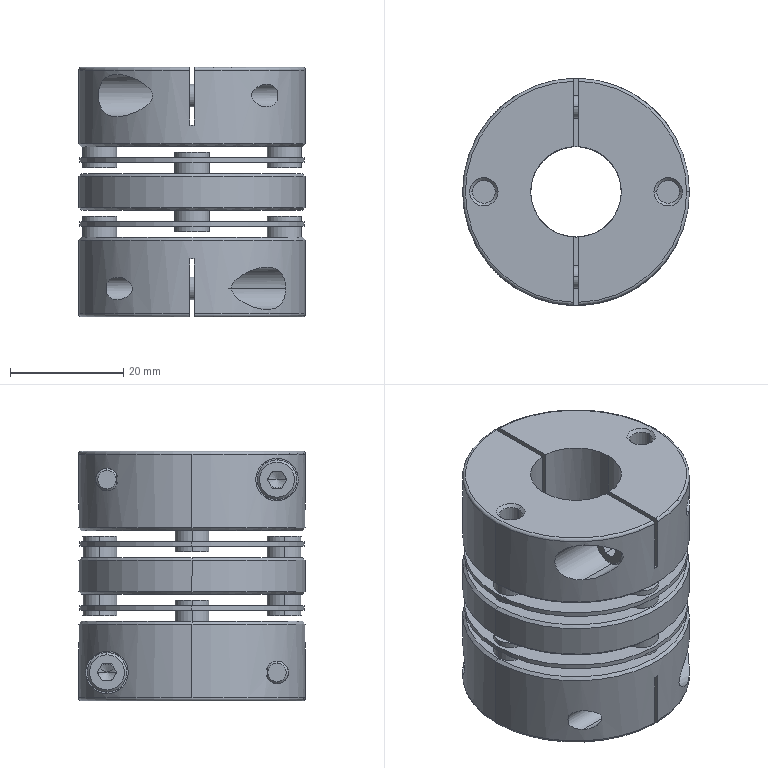Component | SolidWorks | Q1-A12-S21-Q1A.SLDASQ-1_Q1-CPDW40-16-16-1 | 5 solids | 254 faces | volume 34981 mm3 | plane 107 | cylinder 101 | cone 40 | torus 6 | commonest cylinder face diameters 6 x32 4 x24 7 x8 4.5 x8 7.5 x8 21 x6 40 x6 16 x5